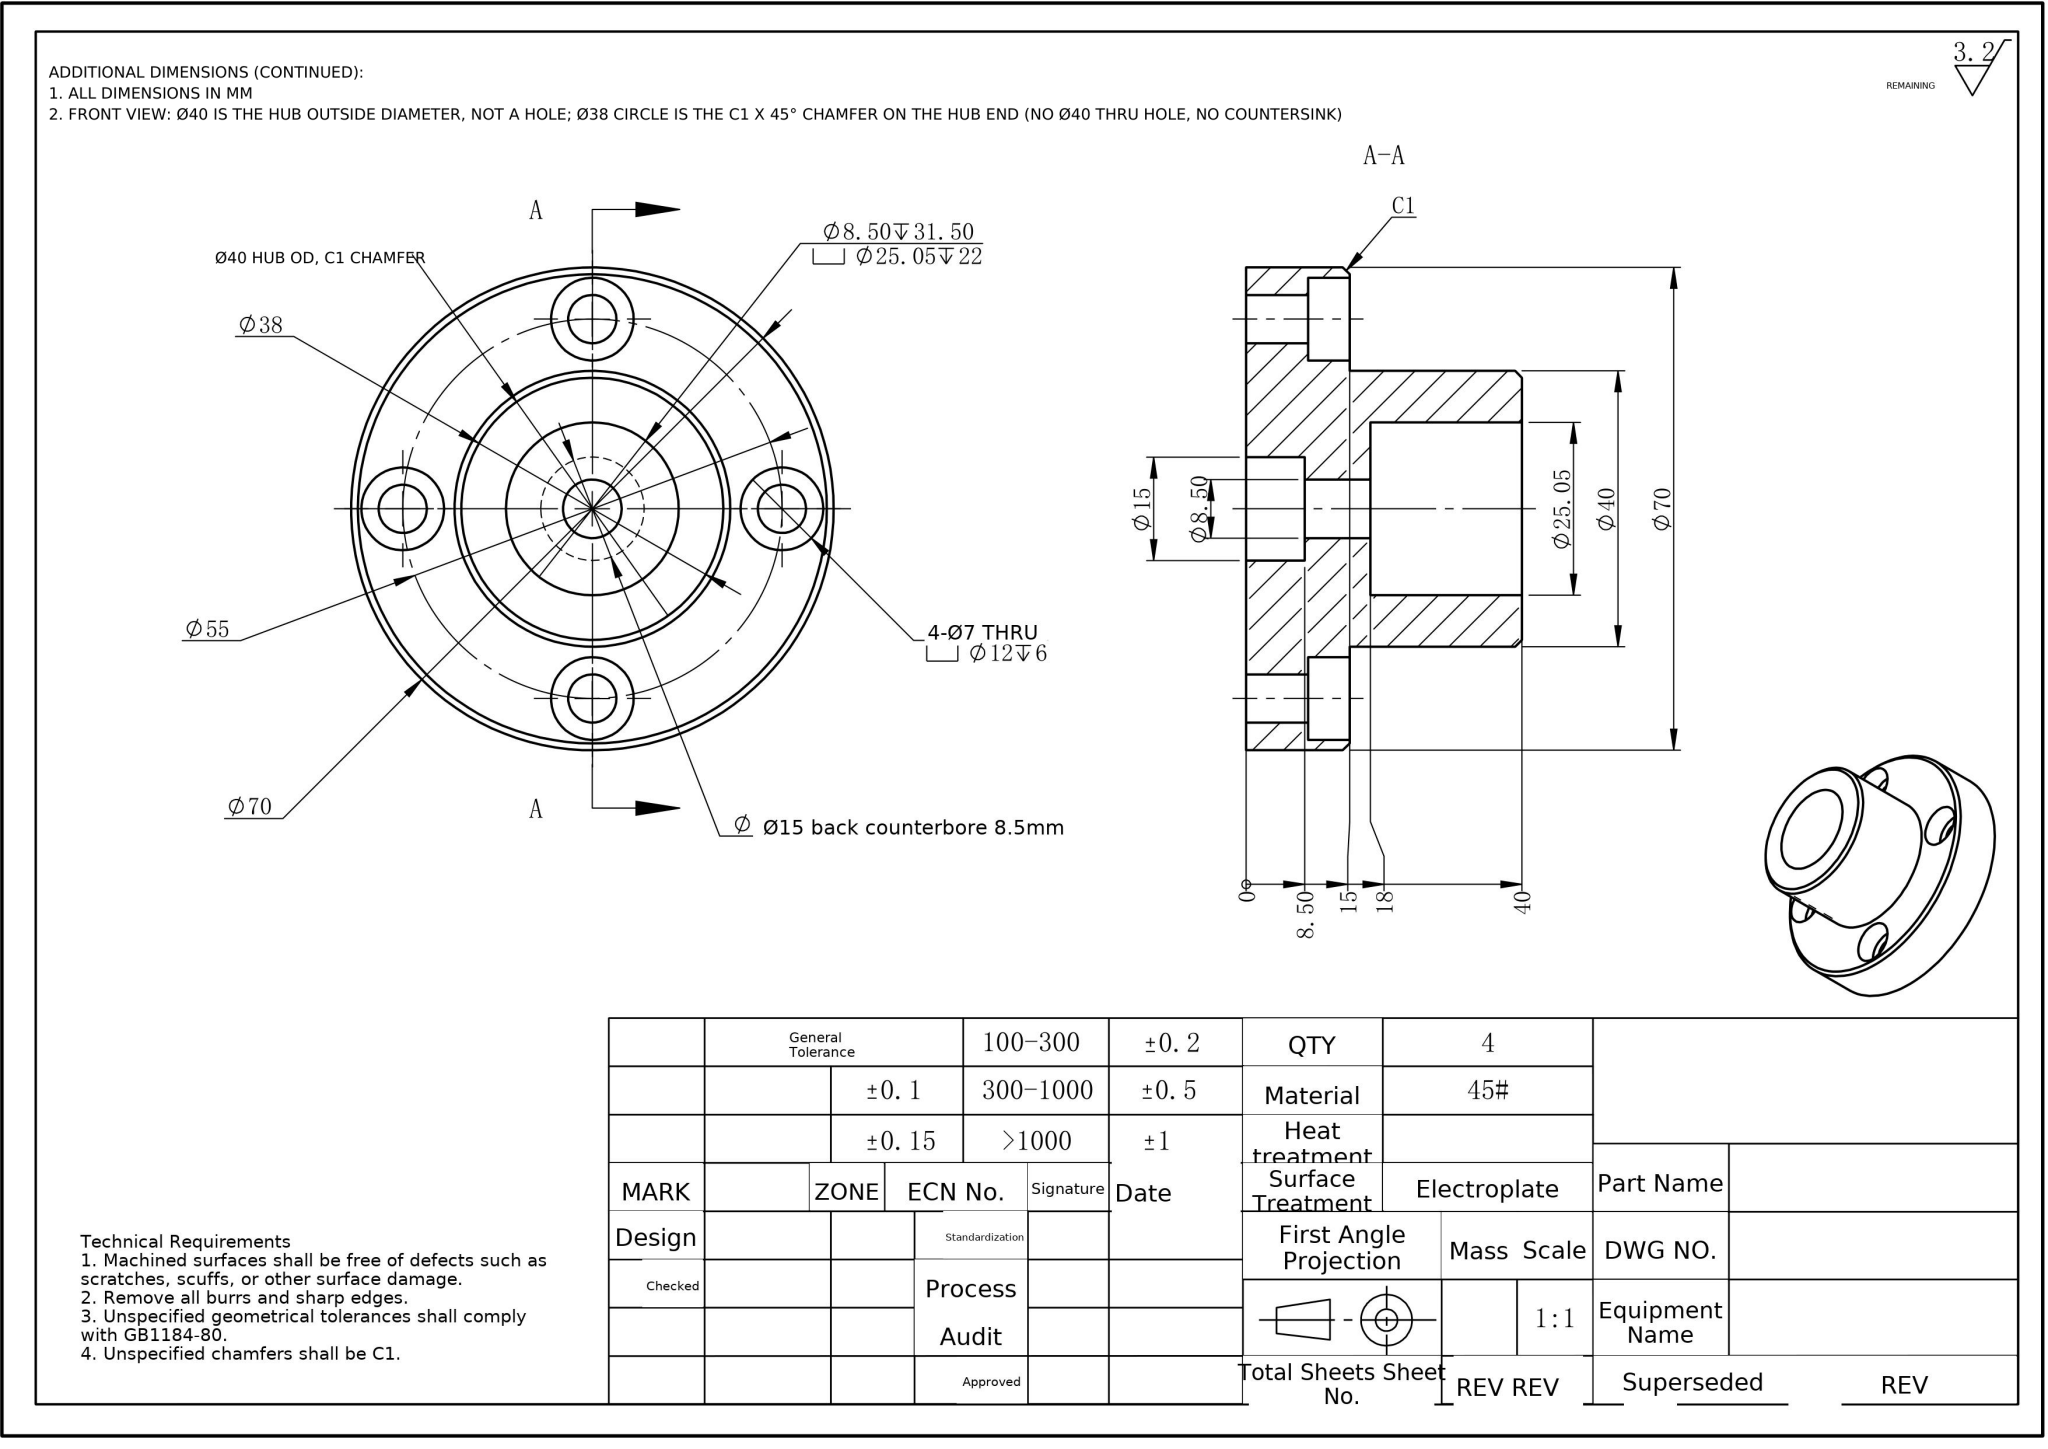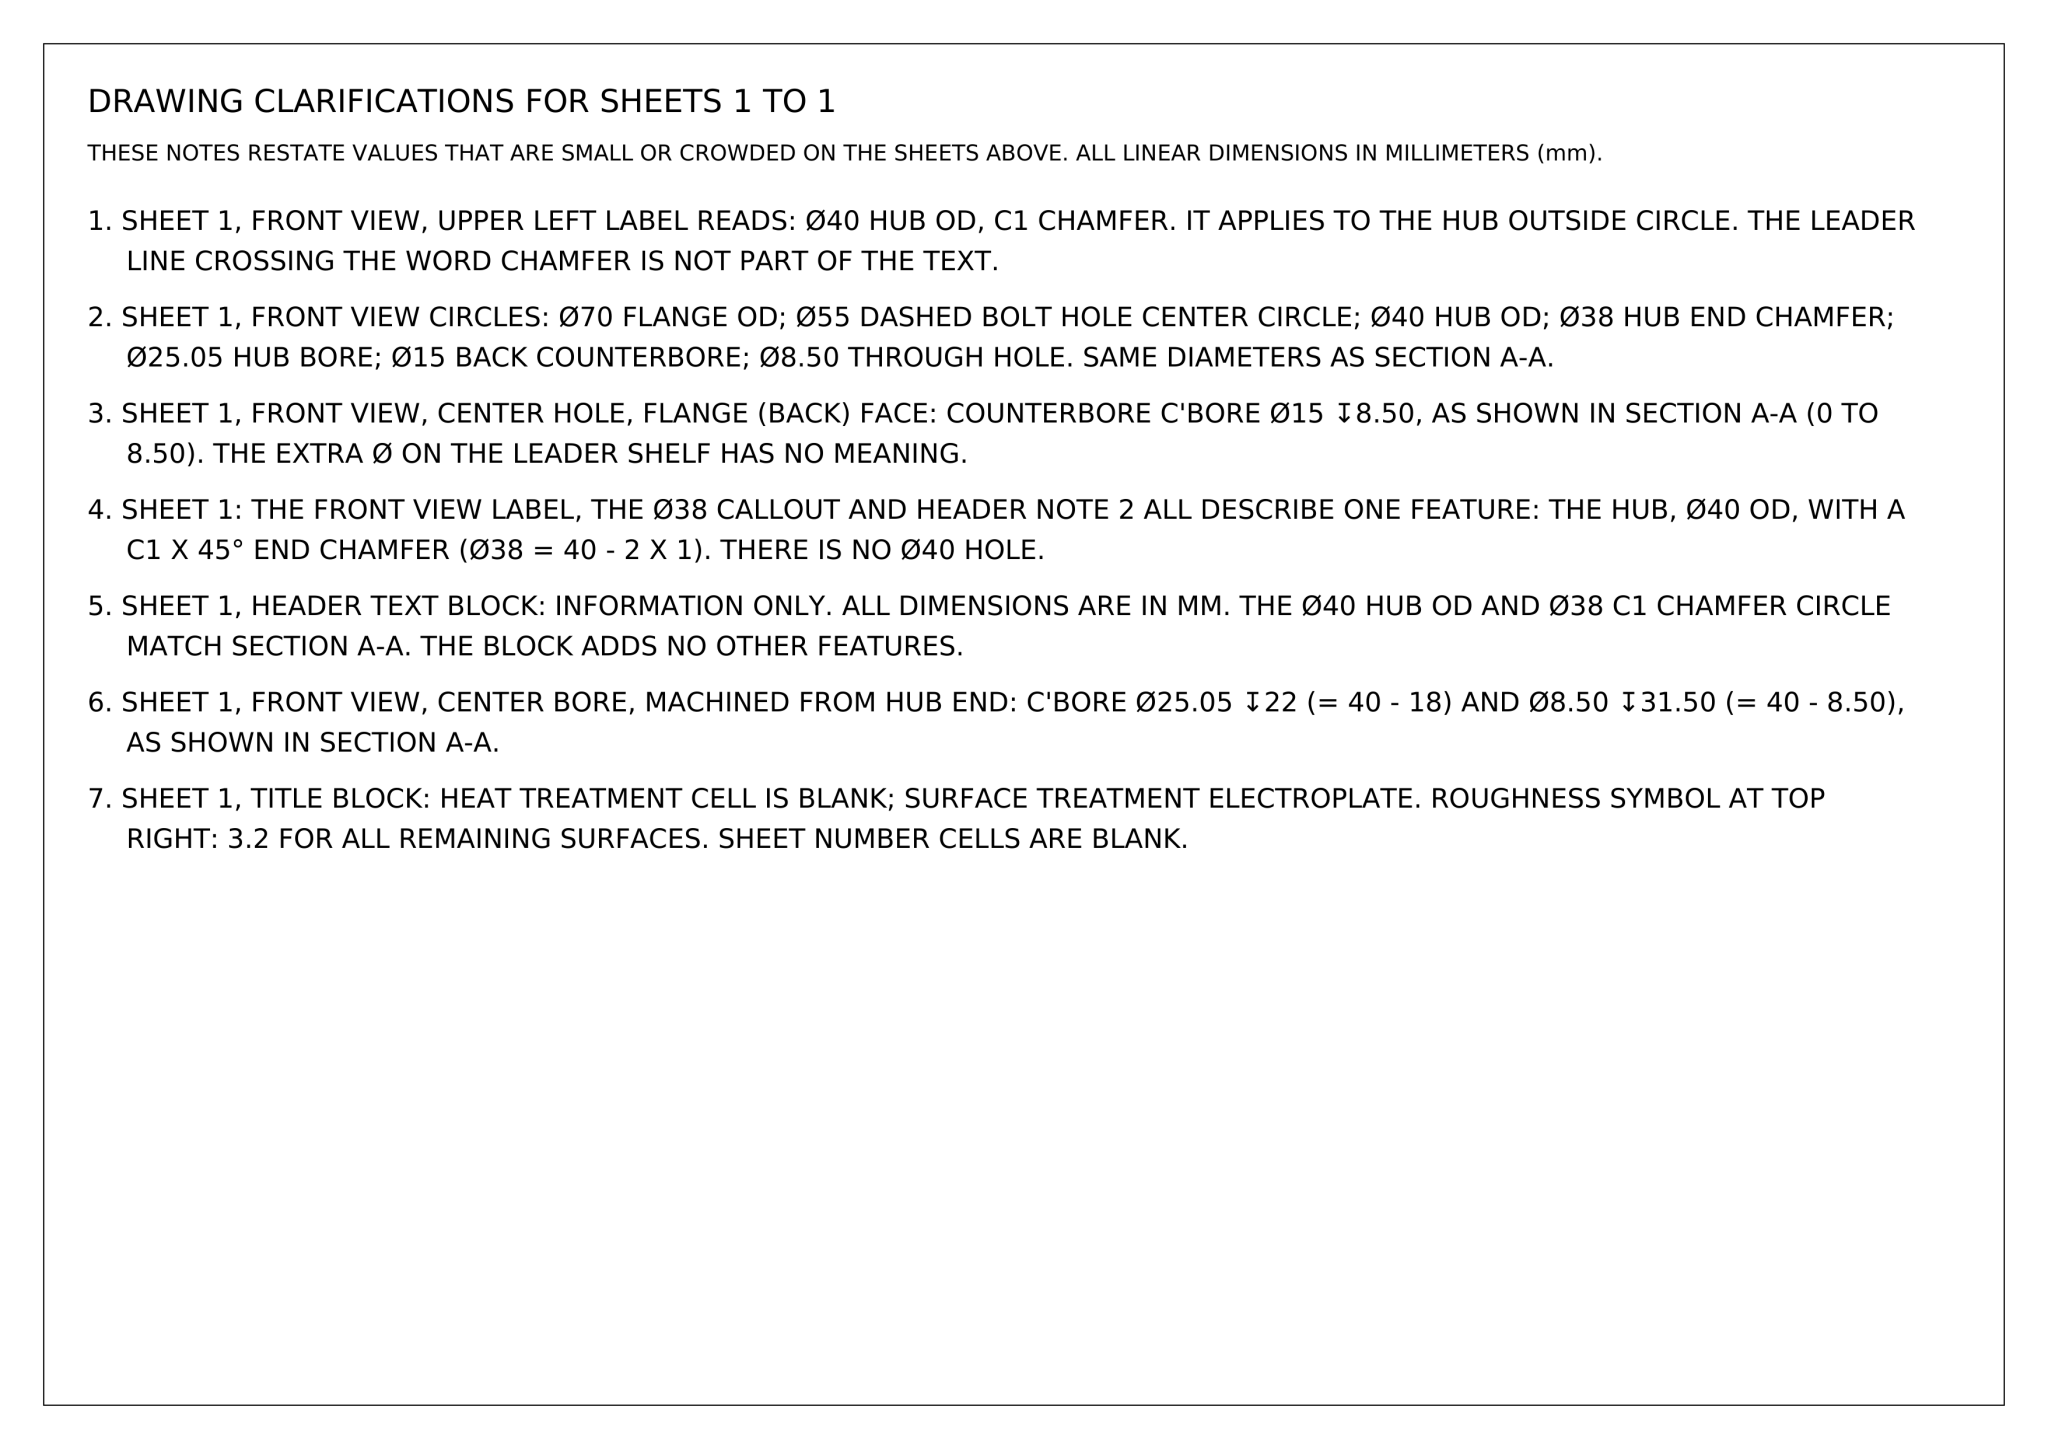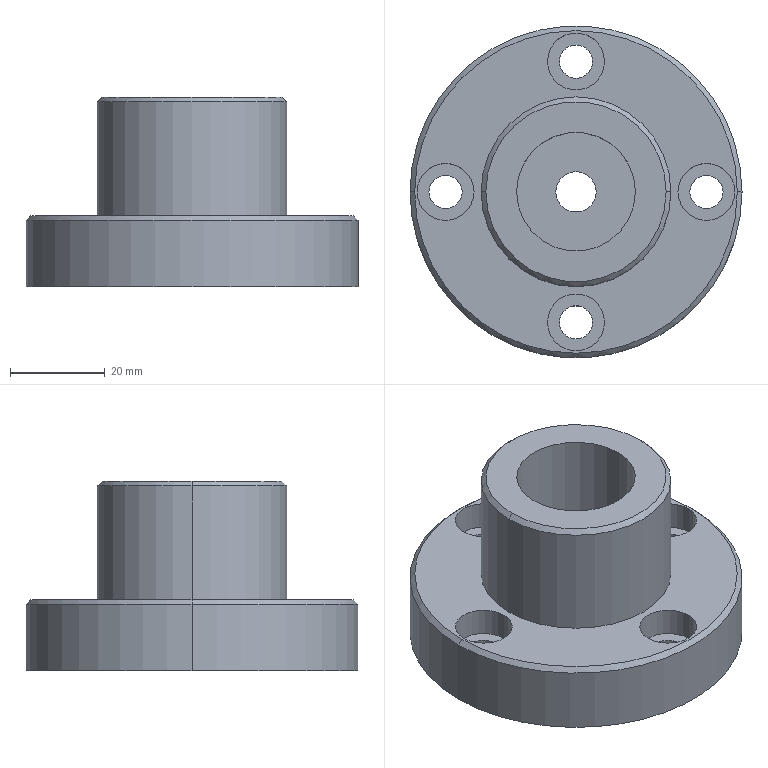Part | NX | mm | 1 solid | 39 faces | box 70 x 70 x 40 mm | volume 71989 mm3 | cylinder 26 | plane 9 | cone 4 | commonest cylinder face diameters 12 x8 7 x8 15 x2 25.05 x2 40 x2 70 x2 8.5 x2